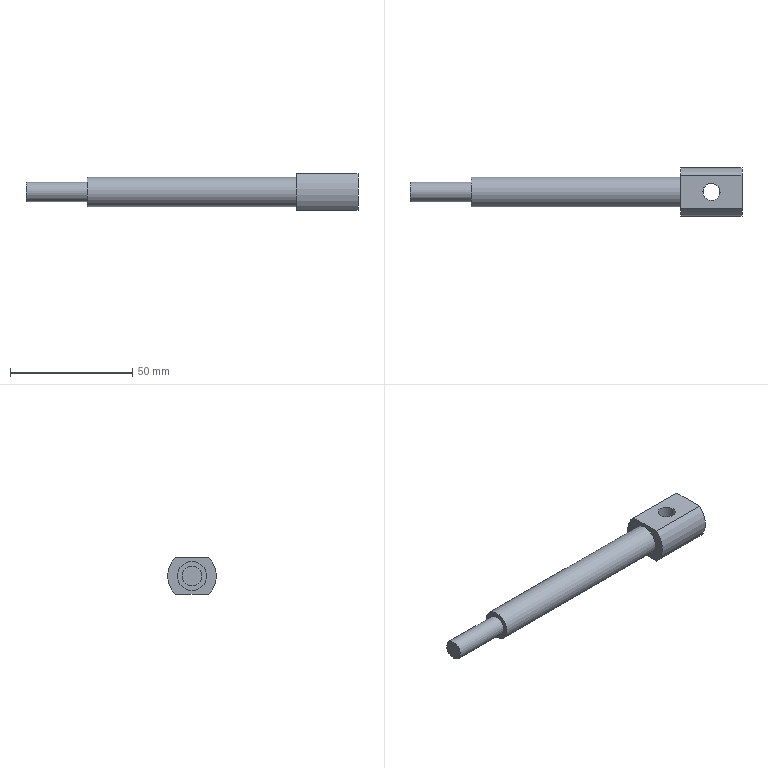Component | NX | LOCKING_SHAFT_2 | 1 solid | 11 faces | box 136 x 20 x 15 mm | volume 17126 mm3 | plane 6 | cylinder 5 | commonest cylinder face diameters 20 x2 12 x1 8 x1 7 x1
STEP:
#1=CARTESIAN_POINT('',(0.,0.,0.));
#2=DIRECTION('',(0.,0.,1.));
#3=DIRECTION('',(1.,0.,0.));
#4=AXIS2_PLACEMENT_3D('',#1,#2,#3);
#5=CARTESIAN_POINT('',(13.092,273.621,195.845));
#6=VERTEX_POINT('',#5);
#7=CARTESIAN_POINT('',(13.092,273.621,201.845));
#8=DIRECTION('',(-1.,0.,0.));
#9=DIRECTION('',(0.,0.,-1.));
#10=AXIS2_PLACEMENT_3D('',#7,#8,#9);
#11=CIRCLE('',#10,6.);
#12=CARTESIAN_POINT('',(13.092,273.621,201.845));
#13=DIRECTION('',(-1.,0.,0.));
#14=DIRECTION('',(0.,0.,-1.));
#15=AXIS2_PLACEMENT_3D('',#12,#13,#14);
#16=PLANE('',#15);
#17=CARTESIAN_POINT('',(0.,0.));
#18=DIRECTION('',(1.,0.));
#19=AXIS2_PLACEMENT_2D('',#17,#18);
#20=CIRCLE('',#19,6.);
#21=(GEOMETRIC_REPRESENTATION_CONTEXT(2)PARAMETRIC_REPRESENTATION_CONTEXT()REPRESENTATION_CONTEXT('',''));
#22=DEFINITIONAL_REPRESENTATION('',(#20),#21);
#23=PCURVE('',#16,#22);
#24=CARTESIAN_POINT('',(13.092,273.621,201.845));
#25=DIRECTION('',(-1.,0.,0.));
#26=DIRECTION('',(0.,0.,-1.));
#27=AXIS2_PLACEMENT_3D('',#24,#25,#26);
#28=CYLINDRICAL_SURFACE('',#27,6.);
#29=CARTESIAN_POINT('',(0.,0.));
#30=DIRECTION('',(1.,0.));
#31=VECTOR('',#30,1.);
#32=LINE('',#29,#31);
#33=(GEOMETRIC_REPRESENTATION_CONTEXT(2)PARAMETRIC_REPRESENTATION_CONTEXT()REPRESENTATION_CONTEXT('',''));
#34=DEFINITIONAL_REPRESENTATION('',(#32),#33);
#35=PCURVE('',#28,#34);
#36=SURFACE_CURVE('',#11,(#23,#35),.PCURVE_S1.);
#37=EDGE_CURVE('',#6,#6,#36,.T.);
#38=ORIENTED_EDGE('',*,*,#37,.F.);
#39=EDGE_LOOP('',(#38));
#40=FACE_BOUND('',#39,.T.);
#41=CARTESIAN_POINT('',(13.092,267.006,209.345));
#42=VERTEX_POINT('',#41);
#43=CARTESIAN_POINT('',(13.092,267.006,194.345));
#44=VERTEX_POINT('',#43);
#45=CARTESIAN_POINT('',(13.092,273.621,201.845));
#46=DIRECTION('',(1.,0.,0.));
#47=DIRECTION('',(0.,0.,-1.));
#48=AXIS2_PLACEMENT_3D('',#45,#46,#47);
#49=CIRCLE('',#48,10.);
#50=CARTESIAN_POINT('',(10.,0.));
#51=CARTESIAN_POINT('',(10.,-17.321));
#52=CARTESIAN_POINT('',(-5.,-8.66));
#53=CARTESIAN_POINT('',(-20.,-0.));
#54=CARTESIAN_POINT('',(-5.,8.66));
#55=CARTESIAN_POINT('',(10.,17.321));
#56=CARTESIAN_POINT('',(10.,0.));
#57=(BOUNDED_CURVE()B_SPLINE_CURVE(2,(#50,#51,#52,#53,#54,#55,#56),.UNSPECIFIED.,.T.,.F.)B_SPLINE_CURVE_WITH_KNOTS((1,2,2,2,2,1),(-2.094,0.,2.094,4.189,6.283,8.378),.UNSPECIFIED.)CURVE()GEOMETRIC_REPRESENTATION_ITEM()RATIONAL_B_SPLINE_CURVE((1.,0.5,1.,0.5,1.,0.5,1.))REPRESENTATION_ITEM(''));
#58=(GEOMETRIC_REPRESENTATION_CONTEXT(2)PARAMETRIC_REPRESENTATION_CONTEXT()REPRESENTATION_CONTEXT('',''));
#59=DEFINITIONAL_REPRESENTATION('',(#57),#58);
#60=PCURVE('',#16,#59);
#61=CARTESIAN_POINT('',(38.092,273.621,201.845));
#62=DIRECTION('',(-1.,0.,0.));
#63=DIRECTION('',(0.,0.,-1.));
#64=AXIS2_PLACEMENT_3D('',#61,#62,#63);
#65=CYLINDRICAL_SURFACE('',#64,10.);
#66=CARTESIAN_POINT('',(6.283,25.));
#67=DIRECTION('',(-1.,0.));
#68=VECTOR('',#67,1.);
#69=LINE('',#66,#68);
#70=(GEOMETRIC_REPRESENTATION_CONTEXT(2)PARAMETRIC_REPRESENTATION_CONTEXT()REPRESENTATION_CONTEXT('',''));
#71=DEFINITIONAL_REPRESENTATION('',(#69),#70);
#72=PCURVE('',#65,#71);
#73=SURFACE_CURVE('',#49,(#60,#72),.PCURVE_S1.);
#74=EDGE_CURVE('',#42,#44,#73,.T.);
#75=ORIENTED_EDGE('',*,*,#74,.F.);
#76=CARTESIAN_POINT('',(13.092,280.235,209.345));
#77=VERTEX_POINT('',#76);
#78=CARTESIAN_POINT('',(13.092,273.621,209.345));
#79=DIRECTION('',(0.,1.,0.));
#80=VECTOR('',#79,1.);
#81=LINE('',#78,#80);
#82=CARTESIAN_POINT('',(-7.5,0.));
#83=DIRECTION('',(0.,-1.));
#84=VECTOR('',#83,1.);
#85=LINE('',#82,#84);
#86=(GEOMETRIC_REPRESENTATION_CONTEXT(2)PARAMETRIC_REPRESENTATION_CONTEXT()REPRESENTATION_CONTEXT('',''));
#87=DEFINITIONAL_REPRESENTATION('',(#85),#86);
#88=PCURVE('',#16,#87);
#89=CARTESIAN_POINT('',(38.092,273.621,209.345));
#90=DIRECTION('',(0.,0.,1.));
#91=DIRECTION('',(-1.,0.,0.));
#92=AXIS2_PLACEMENT_3D('',#89,#90,#91);
#93=PLANE('',#92);
#94=CARTESIAN_POINT('',(25.,0.));
#95=DIRECTION('',(0.,-1.));
#96=VECTOR('',#95,1.);
#97=LINE('',#94,#96);
#98=(GEOMETRIC_REPRESENTATION_CONTEXT(2)PARAMETRIC_REPRESENTATION_CONTEXT()REPRESENTATION_CONTEXT('',''));
#99=DEFINITIONAL_REPRESENTATION('',(#97),#98);
#100=PCURVE('',#93,#99);
#101=SURFACE_CURVE('',#81,(#88,#100),.PCURVE_S1.);
#102=EDGE_CURVE('',#42,#77,#101,.T.);
#103=ORIENTED_EDGE('',*,*,#102,.T.);
#104=CARTESIAN_POINT('',(13.092,280.235,194.345));
#105=VERTEX_POINT('',#104);
#106=CARTESIAN_POINT('',(13.092,273.621,201.845));
#107=DIRECTION('',(1.,0.,0.));
#108=DIRECTION('',(0.,0.,-1.));
#109=AXIS2_PLACEMENT_3D('',#106,#107,#108);
#110=CIRCLE('',#109,10.);
#111=CARTESIAN_POINT('',(10.,0.));
#112=CARTESIAN_POINT('',(10.,-17.321));
#113=CARTESIAN_POINT('',(-5.,-8.66));
#114=CARTESIAN_POINT('',(-20.,-0.));
#115=CARTESIAN_POINT('',(-5.,8.66));
#116=CARTESIAN_POINT('',(10.,17.321));
#117=CARTESIAN_POINT('',(10.,0.));
#118=(BOUNDED_CURVE()B_SPLINE_CURVE(2,(#111,#112,#113,#114,#115,#116,#117),.UNSPECIFIED.,.T.,.F.)B_SPLINE_CURVE_WITH_KNOTS((1,2,2,2,2,1),(-2.094,0.,2.094,4.189,6.283,8.378),.UNSPECIFIED.)CURVE()GEOMETRIC_REPRESENTATION_ITEM()RATIONAL_B_SPLINE_CURVE((1.,0.5,1.,0.5,1.,0.5,1.))REPRESENTATION_ITEM(''));
#119=(GEOMETRIC_REPRESENTATION_CONTEXT(2)PARAMETRIC_REPRESENTATION_CONTEXT()REPRESENTATION_CONTEXT('',''));
#120=DEFINITIONAL_REPRESENTATION('',(#118),#119);
#121=PCURVE('',#16,#120);
#122=CARTESIAN_POINT('',(38.092,273.621,201.845));
#123=DIRECTION('',(-1.,0.,0.));
#124=DIRECTION('',(0.,0.,-1.));
#125=AXIS2_PLACEMENT_3D('',#122,#123,#124);
#126=CYLINDRICAL_SURFACE('',#125,10.);
#127=CARTESIAN_POINT('',(6.283,25.));
#128=DIRECTION('',(-1.,0.));
#129=VECTOR('',#128,1.);
#130=LINE('',#127,#129);
#131=(GEOMETRIC_REPRESENTATION_CONTEXT(2)PARAMETRIC_REPRESENTATION_CONTEXT()REPRESENTATION_CONTEXT('',''));
#132=DEFINITIONAL_REPRESENTATION('',(#130),#131);
#133=PCURVE('',#126,#132);
#134=SURFACE_CURVE('',#110,(#121,#133),.PCURVE_S1.);
#135=EDGE_CURVE('',#105,#77,#134,.T.);
#136=ORIENTED_EDGE('',*,*,#135,.F.);
#137=CARTESIAN_POINT('',(13.092,273.621,194.345));
#138=DIRECTION('',(0.,-1.,0.));
#139=VECTOR('',#138,1.);
#140=LINE('',#137,#139);
#141=CARTESIAN_POINT('',(7.5,0.));
#142=DIRECTION('',(0.,1.));
#143=VECTOR('',#142,1.);
#144=LINE('',#141,#143);
#145=(GEOMETRIC_REPRESENTATION_CONTEXT(2)PARAMETRIC_REPRESENTATION_CONTEXT()REPRESENTATION_CONTEXT('',''));
#146=DEFINITIONAL_REPRESENTATION('',(#144),#145);
#147=PCURVE('',#16,#146);
#148=CARTESIAN_POINT('',(38.092,273.621,194.345));
#149=DIRECTION('',(0.,0.,-1.));
#150=DIRECTION('',(1.,0.,0.));
#151=AXIS2_PLACEMENT_3D('',#148,#149,#150);
#152=PLANE('',#151);
#153=CARTESIAN_POINT('',(-25.,0.));
#154=DIRECTION('',(0.,1.));
#155=VECTOR('',#154,1.);
#156=LINE('',#153,#155);
#157=(GEOMETRIC_REPRESENTATION_CONTEXT(2)PARAMETRIC_REPRESENTATION_CONTEXT()REPRESENTATION_CONTEXT('',''));
#158=DEFINITIONAL_REPRESENTATION('',(#156),#157);
#159=PCURVE('',#152,#158);
#160=SURFACE_CURVE('',#140,(#147,#159),.PCURVE_S1.);
#161=EDGE_CURVE('',#105,#44,#160,.T.);
#162=ORIENTED_EDGE('',*,*,#161,.T.);
#163=EDGE_LOOP('',(#75,#103,#136,#162));
#164=FACE_BOUND('',#163,.T.);
#165=ADVANCED_FACE('',(#40,#164),#16,.T.);
#166=CARTESIAN_POINT('',(38.092,280.235,209.345));
#167=VERTEX_POINT('',#166);
#168=CARTESIAN_POINT('',(38.092,280.235,194.345));
#169=VERTEX_POINT('',#168);
#170=CARTESIAN_POINT('',(38.092,273.621,201.845));
#171=DIRECTION('',(-1.,0.,0.));
#172=DIRECTION('',(0.,0.,-1.));
#173=AXIS2_PLACEMENT_3D('',#170,#171,#172);
#174=CIRCLE('',#173,10.);
#175=CARTESIAN_POINT('',(38.092,273.621,201.845));
#176=DIRECTION('',(1.,0.,0.));
#177=DIRECTION('',(0.,0.,1.));
#178=AXIS2_PLACEMENT_3D('',#175,#176,#177);
#179=PLANE('',#178);
#180=CARTESIAN_POINT('',(-10.,0.));
#181=CARTESIAN_POINT('',(-10.,17.321));
#182=CARTESIAN_POINT('',(5.,8.66));
#183=CARTESIAN_POINT('',(20.,0.));
#184=CARTESIAN_POINT('',(5.,-8.66));
#185=CARTESIAN_POINT('',(-10.,-17.321));
#186=CARTESIAN_POINT('',(-10.,0.));
#187=(BOUNDED_CURVE()B_SPLINE_CURVE(2,(#180,#181,#182,#183,#184,#185,#186),.UNSPECIFIED.,.T.,.F.)B_SPLINE_CURVE_WITH_KNOTS((1,2,2,2,2,1),(-2.094,0.,2.094,4.189,6.283,8.378),.UNSPECIFIED.)CURVE()GEOMETRIC_REPRESENTATION_ITEM()RATIONAL_B_SPLINE_CURVE((1.,0.5,1.,0.5,1.,0.5,1.))REPRESENTATION_ITEM(''));
#188=(GEOMETRIC_REPRESENTATION_CONTEXT(2)PARAMETRIC_REPRESENTATION_CONTEXT()REPRESENTATION_CONTEXT('',''));
#189=DEFINITIONAL_REPRESENTATION('',(#187),#188);
#190=PCURVE('',#179,#189);
#191=CARTESIAN_POINT('',(-0.,0.));
#192=DIRECTION('',(1.,0.));
#193=VECTOR('',#192,1.);
#194=LINE('',#191,#193);
#195=(GEOMETRIC_REPRESENTATION_CONTEXT(2)PARAMETRIC_REPRESENTATION_CONTEXT()REPRESENTATION_CONTEXT('',''));
#196=DEFINITIONAL_REPRESENTATION('',(#194),#195);
#197=PCURVE('',#126,#196);
#198=SURFACE_CURVE('',#174,(#190,#197),.PCURVE_S1.);
#199=EDGE_CURVE('',#167,#169,#198,.T.);
#200=ORIENTED_EDGE('',*,*,#199,.F.);
#201=CARTESIAN_POINT('',(38.092,267.006,209.345));
#202=VERTEX_POINT('',#201);
#203=CARTESIAN_POINT('',(38.092,273.621,209.345));
#204=DIRECTION('',(0.,-1.,0.));
#205=VECTOR('',#204,1.);
#206=LINE('',#203,#205);
#207=CARTESIAN_POINT('',(7.5,0.));
#208=DIRECTION('',(0.,1.));
#209=VECTOR('',#208,1.);
#210=LINE('',#207,#209);
#211=(GEOMETRIC_REPRESENTATION_CONTEXT(2)PARAMETRIC_REPRESENTATION_CONTEXT()REPRESENTATION_CONTEXT('',''));
#212=DEFINITIONAL_REPRESENTATION('',(#210),#211);
#213=PCURVE('',#179,#212);
#214=CARTESIAN_POINT('',(0.,0.));
#215=DIRECTION('',(0.,1.));
#216=VECTOR('',#215,1.);
#217=LINE('',#214,#216);
#218=(GEOMETRIC_REPRESENTATION_CONTEXT(2)PARAMETRIC_REPRESENTATION_CONTEXT()REPRESENTATION_CONTEXT('',''));
#219=DEFINITIONAL_REPRESENTATION('',(#217),#218);
#220=PCURVE('',#93,#219);
#221=SURFACE_CURVE('',#206,(#213,#220),.PCURVE_S1.);
#222=EDGE_CURVE('',#167,#202,#221,.T.);
#223=ORIENTED_EDGE('',*,*,#222,.T.);
#224=CARTESIAN_POINT('',(38.092,267.006,194.345));
#225=VERTEX_POINT('',#224);
#226=CARTESIAN_POINT('',(38.092,273.621,201.845));
#227=DIRECTION('',(-1.,0.,0.));
#228=DIRECTION('',(0.,0.,-1.));
#229=AXIS2_PLACEMENT_3D('',#226,#227,#228);
#230=CIRCLE('',#229,10.);
#231=CARTESIAN_POINT('',(-10.,0.));
#232=CARTESIAN_POINT('',(-10.,17.321));
#233=CARTESIAN_POINT('',(5.,8.66));
#234=CARTESIAN_POINT('',(20.,0.));
#235=CARTESIAN_POINT('',(5.,-8.66));
#236=CARTESIAN_POINT('',(-10.,-17.321));
#237=CARTESIAN_POINT('',(-10.,0.));
#238=(BOUNDED_CURVE()B_SPLINE_CURVE(2,(#231,#232,#233,#234,#235,#236,#237),.UNSPECIFIED.,.T.,.F.)B_SPLINE_CURVE_WITH_KNOTS((1,2,2,2,2,1),(-2.094,0.,2.094,4.189,6.283,8.378),.UNSPECIFIED.)CURVE()GEOMETRIC_REPRESENTATION_ITEM()RATIONAL_B_SPLINE_CURVE((1.,0.5,1.,0.5,1.,0.5,1.))REPRESENTATION_ITEM(''));
#239=(GEOMETRIC_REPRESENTATION_CONTEXT(2)PARAMETRIC_REPRESENTATION_CONTEXT()REPRESENTATION_CONTEXT('',''));
#240=DEFINITIONAL_REPRESENTATION('',(#238),#239);
#241=PCURVE('',#179,#240);
#242=CARTESIAN_POINT('',(0.,0.));
#243=DIRECTION('',(1.,0.));
#244=VECTOR('',#243,1.);
#245=LINE('',#242,#244);
#246=(GEOMETRIC_REPRESENTATION_CONTEXT(2)PARAMETRIC_REPRESENTATION_CONTEXT()REPRESENTATION_CONTEXT('',''));
#247=DEFINITIONAL_REPRESENTATION('',(#245),#246);
#248=PCURVE('',#65,#247);
#249=SURFACE_CURVE('',#230,(#241,#248),.PCURVE_S1.);
#250=EDGE_CURVE('',#225,#202,#249,.T.);
#251=ORIENTED_EDGE('',*,*,#250,.F.);
#252=CARTESIAN_POINT('',(38.092,273.621,194.345));
#253=DIRECTION('',(0.,1.,0.));
#254=VECTOR('',#253,1.);
#255=LINE('',#252,#254);
#256=CARTESIAN_POINT('',(-7.5,0.));
#257=DIRECTION('',(0.,-1.));
#258=VECTOR('',#257,1.);
#259=LINE('',#256,#258);
#260=(GEOMETRIC_REPRESENTATION_CONTEXT(2)PARAMETRIC_REPRESENTATION_CONTEXT()REPRESENTATION_CONTEXT('',''));
#261=DEFINITIONAL_REPRESENTATION('',(#259),#260);
#262=PCURVE('',#179,#261);
#263=CARTESIAN_POINT('',(0.,0.));
#264=DIRECTION('',(0.,-1.));
#265=VECTOR('',#264,1.);
#266=LINE('',#263,#265);
#267=(GEOMETRIC_REPRESENTATION_CONTEXT(2)PARAMETRIC_REPRESENTATION_CONTEXT()REPRESENTATION_CONTEXT('',''));
#268=DEFINITIONAL_REPRESENTATION('',(#266),#267);
#269=PCURVE('',#152,#268);
#270=SURFACE_CURVE('',#255,(#262,#269),.PCURVE_S1.);
#271=EDGE_CURVE('',#225,#169,#270,.T.);
#272=ORIENTED_EDGE('',*,*,#271,.T.);
#273=EDGE_LOOP('',(#200,#223,#251,#272));
#274=FACE_BOUND('',#273,.T.);
#275=ADVANCED_FACE('',(#274),#179,.T.);
#276=ORIENTED_EDGE('',*,*,#135,.T.);
#277=CARTESIAN_POINT('',(38.092,280.235,209.345));
#278=DIRECTION('',(1.,0.,0.));
#279=VECTOR('',#278,1.);
#280=LINE('',#277,#279);
#281=CARTESIAN_POINT('',(3.864,0.));
#282=DIRECTION('',(0.,-1.));
#283=VECTOR('',#282,1.);
#284=LINE('',#281,#283);
#285=(GEOMETRIC_REPRESENTATION_CONTEXT(2)PARAMETRIC_REPRESENTATION_CONTEXT()REPRESENTATION_CONTEXT('',''));
#286=DEFINITIONAL_REPRESENTATION('',(#284),#285);
#287=PCURVE('',#126,#286);
#288=CARTESIAN_POINT('',(0.,-6.614));
#289=DIRECTION('',(-1.,0.));
#290=VECTOR('',#289,1.);
#291=LINE('',#288,#290);
#292=(GEOMETRIC_REPRESENTATION_CONTEXT(2)PARAMETRIC_REPRESENTATION_CONTEXT()REPRESENTATION_CONTEXT('',''));
#293=DEFINITIONAL_REPRESENTATION('',(#291),#292);
#294=PCURVE('',#93,#293);
#295=SURFACE_CURVE('',#280,(#287,#294),.PCURVE_S1.);
#296=EDGE_CURVE('',#77,#167,#295,.T.);
#297=ORIENTED_EDGE('',*,*,#296,.T.);
#298=ORIENTED_EDGE('',*,*,#199,.T.);
#299=CARTESIAN_POINT('',(38.092,280.235,194.345));
#300=DIRECTION('',(-1.,0.,0.));
#301=VECTOR('',#300,1.);
#302=LINE('',#299,#301);
#303=CARTESIAN_POINT('',(5.56,0.));
#304=DIRECTION('',(0.,1.));
#305=VECTOR('',#304,1.);
#306=LINE('',#303,#305);
#307=(GEOMETRIC_REPRESENTATION_CONTEXT(2)PARAMETRIC_REPRESENTATION_CONTEXT()REPRESENTATION_CONTEXT('',''));
#308=DEFINITIONAL_REPRESENTATION('',(#306),#307);
#309=PCURVE('',#126,#308);
#310=CARTESIAN_POINT('',(0.,-6.614));
#311=DIRECTION('',(-1.,0.));
#312=VECTOR('',#311,1.);
#313=LINE('',#310,#312);
#314=(GEOMETRIC_REPRESENTATION_CONTEXT(2)PARAMETRIC_REPRESENTATION_CONTEXT()REPRESENTATION_CONTEXT('',''));
#315=DEFINITIONAL_REPRESENTATION('',(#313),#314);
#316=PCURVE('',#152,#315);
#317=SURFACE_CURVE('',#302,(#309,#316),.PCURVE_S1.);
#318=EDGE_CURVE('',#169,#105,#317,.T.);
#319=ORIENTED_EDGE('',*,*,#318,.T.);
#320=EDGE_LOOP('',(#276,#297,#298,#319));
#321=FACE_BOUND('',#320,.T.);
#322=ADVANCED_FACE('',(#321),#126,.T.);
#323=ORIENTED_EDGE('',*,*,#250,.T.);
#324=CARTESIAN_POINT('',(38.092,267.006,209.345));
#325=DIRECTION('',(-1.,0.,0.));
#326=VECTOR('',#325,1.);
#327=LINE('',#324,#326);
#328=CARTESIAN_POINT('',(2.419,0.));
#329=DIRECTION('',(0.,1.));
#330=VECTOR('',#329,1.);
#331=LINE('',#328,#330);
#332=(GEOMETRIC_REPRESENTATION_CONTEXT(2)PARAMETRIC_REPRESENTATION_CONTEXT()REPRESENTATION_CONTEXT('',''));
#333=DEFINITIONAL_REPRESENTATION('',(#331),#332);
#334=PCURVE('',#65,#333);
#335=CARTESIAN_POINT('',(0.,6.614));
#336=DIRECTION('',(1.,0.));
#337=VECTOR('',#336,1.);
#338=LINE('',#335,#337);
#339=(GEOMETRIC_REPRESENTATION_CONTEXT(2)PARAMETRIC_REPRESENTATION_CONTEXT()REPRESENTATION_CONTEXT('',''));
#340=DEFINITIONAL_REPRESENTATION('',(#338),#339);
#341=PCURVE('',#93,#340);
#342=SURFACE_CURVE('',#327,(#334,#341),.PCURVE_S1.);
#343=EDGE_CURVE('',#202,#42,#342,.T.);
#344=ORIENTED_EDGE('',*,*,#343,.T.);
#345=ORIENTED_EDGE('',*,*,#74,.T.);
#346=CARTESIAN_POINT('',(38.092,267.006,194.345));
#347=DIRECTION('',(1.,0.,0.));
#348=VECTOR('',#347,1.);
#349=LINE('',#346,#348);
#350=CARTESIAN_POINT('',(0.7227,0.));
#351=DIRECTION('',(0.,-1.));
#352=VECTOR('',#351,1.);
#353=LINE('',#350,#352);
#354=(GEOMETRIC_REPRESENTATION_CONTEXT(2)PARAMETRIC_REPRESENTATION_CONTEXT()REPRESENTATION_CONTEXT('',''));
#355=DEFINITIONAL_REPRESENTATION('',(#353),#354);
#356=PCURVE('',#65,#355);
#357=CARTESIAN_POINT('',(0.,6.614));
#358=DIRECTION('',(1.,0.));
#359=VECTOR('',#358,1.);
#360=LINE('',#357,#359);
#361=(GEOMETRIC_REPRESENTATION_CONTEXT(2)PARAMETRIC_REPRESENTATION_CONTEXT()REPRESENTATION_CONTEXT('',''));
#362=DEFINITIONAL_REPRESENTATION('',(#360),#361);
#363=PCURVE('',#152,#362);
#364=SURFACE_CURVE('',#349,(#356,#363),.PCURVE_S1.);
#365=EDGE_CURVE('',#44,#225,#364,.T.);
#366=ORIENTED_EDGE('',*,*,#365,.T.);
#367=EDGE_LOOP('',(#323,#344,#345,#366));
#368=FACE_BOUND('',#367,.T.);
#369=ADVANCED_FACE('',(#368),#65,.T.);
#370=CARTESIAN_POINT('',(25.592,270.121,194.345));
#371=VERTEX_POINT('',#370);
#372=CARTESIAN_POINT('',(25.592,273.621,194.345));
#373=DIRECTION('',(0.,0.,-1.));
#374=DIRECTION('',(0.,-1.,0.));
#375=AXIS2_PLACEMENT_3D('',#372,#373,#374);
#376=CIRCLE('',#375,3.5);
#377=CARTESIAN_POINT('',(-12.5,0.));
#378=DIRECTION('',(0.,1.));
#379=AXIS2_PLACEMENT_2D('',#377,#378);
#380=CIRCLE('',#379,3.5);
#381=(GEOMETRIC_REPRESENTATION_CONTEXT(2)PARAMETRIC_REPRESENTATION_CONTEXT()REPRESENTATION_CONTEXT('',''));
#382=DEFINITIONAL_REPRESENTATION('',(#380),#381);
#383=PCURVE('',#152,#382);
#384=CARTESIAN_POINT('',(25.592,273.621,211.345));
#385=DIRECTION('',(0.,0.,-1.));
#386=DIRECTION('',(1.,0.,0.));
#387=AXIS2_PLACEMENT_3D('',#384,#385,#386);
#388=CYLINDRICAL_SURFACE('',#387,3.5);
#389=CARTESIAN_POINT('',(1.571,17.));
#390=DIRECTION('',(1.,0.));
#391=VECTOR('',#390,1.);
#392=LINE('',#389,#391);
#393=(GEOMETRIC_REPRESENTATION_CONTEXT(2)PARAMETRIC_REPRESENTATION_CONTEXT()REPRESENTATION_CONTEXT('',''));
#394=DEFINITIONAL_REPRESENTATION('',(#392),#393);
#395=PCURVE('',#388,#394);
#396=SURFACE_CURVE('',#376,(#383,#395),.PCURVE_S1.);
#397=EDGE_CURVE('',#371,#371,#396,.T.);
#398=ORIENTED_EDGE('',*,*,#397,.F.);
#399=EDGE_LOOP('',(#398));
#400=FACE_BOUND('',#399,.T.);
#401=ORIENTED_EDGE('',*,*,#365,.F.);
#402=ORIENTED_EDGE('',*,*,#161,.F.);
#403=ORIENTED_EDGE('',*,*,#318,.F.);
#404=ORIENTED_EDGE('',*,*,#271,.F.);
#405=EDGE_LOOP('',(#401,#402,#403,#404));
#406=FACE_BOUND('',#405,.T.);
#407=ADVANCED_FACE('',(#400,#406),#152,.T.);
#408=CARTESIAN_POINT('',(22.092,273.621,209.345));
#409=VERTEX_POINT('',#408);
#410=CARTESIAN_POINT('',(25.592,270.121,209.345));
#411=VERTEX_POINT('',#410);
#412=CARTESIAN_POINT('',(25.592,273.621,209.345));
#413=DIRECTION('',(0.,0.,1.));
#414=DIRECTION('',(-1.,0.,0.));
#415=AXIS2_PLACEMENT_3D('',#412,#413,#414);
#416=CIRCLE('',#415,3.5);
#417=CARTESIAN_POINT('',(12.5,0.));
#418=DIRECTION('',(1.,0.));
#419=AXIS2_PLACEMENT_2D('',#417,#418);
#420=CIRCLE('',#419,3.5);
#421=(GEOMETRIC_REPRESENTATION_CONTEXT(2)PARAMETRIC_REPRESENTATION_CONTEXT()REPRESENTATION_CONTEXT('',''));
#422=DEFINITIONAL_REPRESENTATION('',(#420),#421);
#423=PCURVE('',#93,#422);
#424=CARTESIAN_POINT('',(3.142,2.));
#425=DIRECTION('',(-1.,0.));
#426=VECTOR('',#425,1.);
#427=LINE('',#424,#426);
#428=(GEOMETRIC_REPRESENTATION_CONTEXT(2)PARAMETRIC_REPRESENTATION_CONTEXT()REPRESENTATION_CONTEXT('',''));
#429=DEFINITIONAL_REPRESENTATION('',(#427),#428);
#430=PCURVE('',#388,#429);
#431=SURFACE_CURVE('',#416,(#423,#430),.PCURVE_S1.);
#432=EDGE_CURVE('',#409,#411,#431,.T.);
#433=ORIENTED_EDGE('',*,*,#432,.F.);
#434=CARTESIAN_POINT('',(25.592,273.621,209.345));
#435=DIRECTION('',(0.,0.,1.));
#436=DIRECTION('',(-1.,0.,0.));
#437=AXIS2_PLACEMENT_3D('',#434,#435,#436);
#438=CIRCLE('',#437,3.5);
#439=CARTESIAN_POINT('',(12.5,0.));
#440=DIRECTION('',(1.,0.));
#441=AXIS2_PLACEMENT_2D('',#439,#440);
#442=CIRCLE('',#441,3.5);
#443=(GEOMETRIC_REPRESENTATION_CONTEXT(2)PARAMETRIC_REPRESENTATION_CONTEXT()REPRESENTATION_CONTEXT('',''));
#444=DEFINITIONAL_REPRESENTATION('',(#442),#443);
#445=PCURVE('',#93,#444);
#446=CARTESIAN_POINT('',(9.425,2.));
#447=DIRECTION('',(-1.,0.));
#448=VECTOR('',#447,1.);
#449=LINE('',#446,#448);
#450=(GEOMETRIC_REPRESENTATION_CONTEXT(2)PARAMETRIC_REPRESENTATION_CONTEXT()REPRESENTATION_CONTEXT('',''));
#451=DEFINITIONAL_REPRESENTATION('',(#449),#450);
#452=PCURVE('',#388,#451);
#453=SURFACE_CURVE('',#438,(#445,#452),.PCURVE_S1.);
#454=EDGE_CURVE('',#411,#409,#453,.T.);
#455=ORIENTED_EDGE('',*,*,#454,.F.);
#456=EDGE_LOOP('',(#433,#455));
#457=FACE_BOUND('',#456,.T.);
#458=ORIENTED_EDGE('',*,*,#296,.F.);
#459=ORIENTED_EDGE('',*,*,#102,.F.);
#460=ORIENTED_EDGE('',*,*,#343,.F.);
#461=ORIENTED_EDGE('',*,*,#222,.F.);
#462=EDGE_LOOP('',(#458,#459,#460,#461));
#463=FACE_BOUND('',#462,.T.);
#464=ADVANCED_FACE('',(#457,#463),#93,.T.);
#465=CARTESIAN_POINT('',(-72.908,273.621,197.845));
#466=VERTEX_POINT('',#465);
#467=CARTESIAN_POINT('',(-72.908,273.621,201.845));
#468=DIRECTION('',(-1.,0.,0.));
#469=DIRECTION('',(0.,0.,-1.));
#470=AXIS2_PLACEMENT_3D('',#467,#468,#469);
#471=CIRCLE('',#470,4.);
#472=CARTESIAN_POINT('',(-72.908,273.621,201.845));
#473=DIRECTION('',(-1.,0.,0.));
#474=DIRECTION('',(0.,0.,-1.));
#475=AXIS2_PLACEMENT_3D('',#472,#473,#474);
#476=PLANE('',#475);
#477=CARTESIAN_POINT('',(0.,0.));
#478=DIRECTION('',(1.,0.));
#479=AXIS2_PLACEMENT_2D('',#477,#478);
#480=CIRCLE('',#479,4.);
#481=(GEOMETRIC_REPRESENTATION_CONTEXT(2)PARAMETRIC_REPRESENTATION_CONTEXT()REPRESENTATION_CONTEXT('',''));
#482=DEFINITIONAL_REPRESENTATION('',(#480),#481);
#483=PCURVE('',#476,#482);
#484=CARTESIAN_POINT('',(-72.908,273.621,201.845));
#485=DIRECTION('',(-1.,0.,0.));
#486=DIRECTION('',(0.,0.,-1.));
#487=AXIS2_PLACEMENT_3D('',#484,#485,#486);
#488=CYLINDRICAL_SURFACE('',#487,4.);
#489=CARTESIAN_POINT('',(0.,0.));
#490=DIRECTION('',(1.,0.));
#491=VECTOR('',#490,1.);
#492=LINE('',#489,#491);
#493=(GEOMETRIC_REPRESENTATION_CONTEXT(2)PARAMETRIC_REPRESENTATION_CONTEXT()REPRESENTATION_CONTEXT('',''));
#494=DEFINITIONAL_REPRESENTATION('',(#492),#493);
#495=PCURVE('',#488,#494);
#496=SURFACE_CURVE('',#471,(#483,#495),.PCURVE_S1.);
#497=EDGE_CURVE('',#466,#466,#496,.T.);
#498=ORIENTED_EDGE('',*,*,#497,.F.);
#499=EDGE_LOOP('',(#498));
#500=FACE_BOUND('',#499,.T.);
#501=CARTESIAN_POINT('',(-72.908,273.621,195.845));
#502=VERTEX_POINT('',#501);
#503=CARTESIAN_POINT('',(-72.908,273.621,201.845));
#504=DIRECTION('',(1.,0.,0.));
#505=DIRECTION('',(0.,0.,-1.));
#506=AXIS2_PLACEMENT_3D('',#503,#504,#505);
#507=CIRCLE('',#506,6.);
#508=CARTESIAN_POINT('',(6.,0.));
#509=CARTESIAN_POINT('',(6.,-10.392));
#510=CARTESIAN_POINT('',(-3.,-5.196));
#511=CARTESIAN_POINT('',(-12.,-0.));
#512=CARTESIAN_POINT('',(-3.,5.196));
#513=CARTESIAN_POINT('',(6.,10.392));
#514=CARTESIAN_POINT('',(6.,0.));
#515=(BOUNDED_CURVE()B_SPLINE_CURVE(2,(#508,#509,#510,#511,#512,#513,#514),.UNSPECIFIED.,.T.,.F.)B_SPLINE_CURVE_WITH_KNOTS((1,2,2,2,2,1),(-2.094,0.,2.094,4.189,6.283,8.378),.UNSPECIFIED.)CURVE()GEOMETRIC_REPRESENTATION_ITEM()RATIONAL_B_SPLINE_CURVE((1.,0.5,1.,0.5,1.,0.5,1.))REPRESENTATION_ITEM(''));
#516=(GEOMETRIC_REPRESENTATION_CONTEXT(2)PARAMETRIC_REPRESENTATION_CONTEXT()REPRESENTATION_CONTEXT('',''));
#517=DEFINITIONAL_REPRESENTATION('',(#515),#516);
#518=PCURVE('',#476,#517);
#519=CARTESIAN_POINT('',(6.283,86.));
#520=DIRECTION('',(-1.,0.));
#521=VECTOR('',#520,1.);
#522=LINE('',#519,#521);
#523=(GEOMETRIC_REPRESENTATION_CONTEXT(2)PARAMETRIC_REPRESENTATION_CONTEXT()REPRESENTATION_CONTEXT('',''));
#524=DEFINITIONAL_REPRESENTATION('',(#522),#523);
#525=PCURVE('',#28,#524);
#526=SURFACE_CURVE('',#507,(#518,#525),.PCURVE_S1.);
#527=EDGE_CURVE('',#502,#502,#526,.T.);
#528=ORIENTED_EDGE('',*,*,#527,.F.);
#529=EDGE_LOOP('',(#528));
#530=FACE_BOUND('',#529,.T.);
#531=ADVANCED_FACE('',(#500,#530),#476,.T.);
#532=ORIENTED_EDGE('',*,*,#527,.T.);
#533=CARTESIAN_POINT('',(13.092,273.621,195.845));
#534=CARTESIAN_POINT('',(-72.908,273.621,195.845));
#535=B_SPLINE_CURVE_WITH_KNOTS('',1,(#533,#534),.UNSPECIFIED.,.F.,.F.,(2,2),(0.,86.),.PIECEWISE_BEZIER_KNOTS.);
#536=CARTESIAN_POINT('',(0.,0.));
#537=DIRECTION('',(0.,1.));
#538=VECTOR('',#537,1.);
#539=LINE('',#536,#538);
#540=(GEOMETRIC_REPRESENTATION_CONTEXT(2)PARAMETRIC_REPRESENTATION_CONTEXT()REPRESENTATION_CONTEXT('',''));
#541=DEFINITIONAL_REPRESENTATION('',(#539),#540);
#542=PCURVE('',#28,#541);
#543=CARTESIAN_POINT('',(6.283,0.));
#544=DIRECTION('',(0.,1.));
#545=VECTOR('',#544,1.);
#546=LINE('',#543,#545);
#547=(GEOMETRIC_REPRESENTATION_CONTEXT(2)PARAMETRIC_REPRESENTATION_CONTEXT()REPRESENTATION_CONTEXT('',''));
#548=DEFINITIONAL_REPRESENTATION('',(#546),#547);
#549=PCURVE('',#28,#548);
#550=SEAM_CURVE('',#535,(#542,#549),.PCURVE_S1.);
#551=EDGE_CURVE('',#6,#502,#550,.T.);
#552=ORIENTED_EDGE('',*,*,#551,.F.);
#553=ORIENTED_EDGE('',*,*,#37,.T.);
#554=ORIENTED_EDGE('',*,*,#551,.T.);
#555=EDGE_LOOP('',(#532,#552,#553,#554));
#556=FACE_BOUND('',#555,.T.);
#557=ADVANCED_FACE('',(#556),#28,.T.);
#558=CARTESIAN_POINT('',(-97.908,273.621,197.845));
#559=VERTEX_POINT('',#558);
#560=CARTESIAN_POINT('',(-97.908,273.621,201.845));
#561=DIRECTION('',(1.,0.,0.));
#562=DIRECTION('',(0.,0.,-1.));
#563=AXIS2_PLACEMENT_3D('',#560,#561,#562);
#564=CIRCLE('',#563,4.);
#565=CARTESIAN_POINT('',(-97.908,273.621,201.845));
#566=DIRECTION('',(-1.,0.,0.));
#567=DIRECTION('',(0.,0.,-1.));
#568=AXIS2_PLACEMENT_3D('',#565,#566,#567);
#569=PLANE('',#568);
#570=CARTESIAN_POINT('',(4.,0.));
#571=CARTESIAN_POINT('',(4.,-6.928));
#572=CARTESIAN_POINT('',(-2.,-3.464));
#573=CARTESIAN_POINT('',(-8.,-0.));
#574=CARTESIAN_POINT('',(-2.,3.464));
#575=CARTESIAN_POINT('',(4.,6.928));
#576=CARTESIAN_POINT('',(4.,0.));
#577=(BOUNDED_CURVE()B_SPLINE_CURVE(2,(#570,#571,#572,#573,#574,#575,#576),.UNSPECIFIED.,.T.,.F.)B_SPLINE_CURVE_WITH_KNOTS((1,2,2,2,2,1),(-2.094,0.,2.094,4.189,6.283,8.378),.UNSPECIFIED.)CURVE()GEOMETRIC_REPRESENTATION_ITEM()RATIONAL_B_SPLINE_CURVE((1.,0.5,1.,0.5,1.,0.5,1.))REPRESENTATION_ITEM(''));
#578=(GEOMETRIC_REPRESENTATION_CONTEXT(2)PARAMETRIC_REPRESENTATION_CONTEXT()REPRESENTATION_CONTEXT('',''));
#579=DEFINITIONAL_REPRESENTATION('',(#577),#578);
#580=PCURVE('',#569,#579);
#581=CARTESIAN_POINT('',(6.283,25.));
#582=DIRECTION('',(-1.,0.));
#583=VECTOR('',#582,1.);
#584=LINE('',#581,#583);
#585=(GEOMETRIC_REPRESENTATION_CONTEXT(2)PARAMETRIC_REPRESENTATION_CONTEXT()REPRESENTATION_CONTEXT('',''));
#586=DEFINITIONAL_REPRESENTATION('',(#584),#585);
#587=PCURVE('',#488,#586);
#588=SURFACE_CURVE('',#564,(#580,#587),.PCURVE_S1.);
#589=EDGE_CURVE('',#559,#559,#588,.T.);
#590=ORIENTED_EDGE('',*,*,#589,.F.);
#591=EDGE_LOOP('',(#590));
#592=FACE_BOUND('',#591,.T.);
#593=ADVANCED_FACE('',(#592),#569,.T.);
#594=ORIENTED_EDGE('',*,*,#589,.T.);
#595=CARTESIAN_POINT('',(-72.908,273.621,197.845));
#596=CARTESIAN_POINT('',(-97.908,273.621,197.845));
#597=B_SPLINE_CURVE_WITH_KNOTS('',1,(#595,#596),.UNSPECIFIED.,.F.,.F.,(2,2),(0.,25.),.PIECEWISE_BEZIER_KNOTS.);
#598=CARTESIAN_POINT('',(0.,0.));
#599=DIRECTION('',(0.,1.));
#600=VECTOR('',#599,1.);
#601=LINE('',#598,#600);
#602=(GEOMETRIC_REPRESENTATION_CONTEXT(2)PARAMETRIC_REPRESENTATION_CONTEXT()REPRESENTATION_CONTEXT('',''));
#603=DEFINITIONAL_REPRESENTATION('',(#601),#602);
#604=PCURVE('',#488,#603);
#605=CARTESIAN_POINT('',(6.283,0.));
#606=DIRECTION('',(0.,1.));
#607=VECTOR('',#606,1.);
#608=LINE('',#605,#607);
#609=(GEOMETRIC_REPRESENTATION_CONTEXT(2)PARAMETRIC_REPRESENTATION_CONTEXT()REPRESENTATION_CONTEXT('',''));
#610=DEFINITIONAL_REPRESENTATION('',(#608),#609);
#611=PCURVE('',#488,#610);
#612=SEAM_CURVE('',#597,(#604,#611),.PCURVE_S1.);
#613=EDGE_CURVE('',#466,#559,#612,.T.);
#614=ORIENTED_EDGE('',*,*,#613,.F.);
#615=ORIENTED_EDGE('',*,*,#497,.T.);
#616=ORIENTED_EDGE('',*,*,#613,.T.);
#617=EDGE_LOOP('',(#594,#614,#615,#616));
#618=FACE_BOUND('',#617,.T.);
#619=ADVANCED_FACE('',(#618),#488,.T.);
#620=ORIENTED_EDGE('',*,*,#454,.F.);
#621=CARTESIAN_POINT('',(25.592,270.121,209.345));
#622=CARTESIAN_POINT('',(25.592,270.121,194.345));
#623=B_SPLINE_CURVE_WITH_KNOTS('',1,(#621,#622),.UNSPECIFIED.,.F.,.F.,(2,2),(2.,17.),.PIECEWISE_BEZIER_KNOTS.);
#624=CARTESIAN_POINT('',(7.854,0.));
#625=DIRECTION('',(0.,1.));
#626=VECTOR('',#625,1.);
#627=LINE('',#624,#626);
#628=(GEOMETRIC_REPRESENTATION_CONTEXT(2)PARAMETRIC_REPRESENTATION_CONTEXT()REPRESENTATION_CONTEXT('',''));
#629=DEFINITIONAL_REPRESENTATION('',(#627),#628);
#630=PCURVE('',#388,#629);
#631=CARTESIAN_POINT('',(1.571,0.));
#632=DIRECTION('',(0.,1.));
#633=VECTOR('',#632,1.);
#634=LINE('',#631,#633);
#635=(GEOMETRIC_REPRESENTATION_CONTEXT(2)PARAMETRIC_REPRESENTATION_CONTEXT()REPRESENTATION_CONTEXT('',''));
#636=DEFINITIONAL_REPRESENTATION('',(#634),#635);
#637=PCURVE('',#388,#636);
#638=SEAM_CURVE('',#623,(#630,#637),.PCURVE_S1.);
#639=EDGE_CURVE('',#411,#371,#638,.T.);
#640=ORIENTED_EDGE('',*,*,#639,.T.);
#641=ORIENTED_EDGE('',*,*,#397,.F.);
#642=ORIENTED_EDGE('',*,*,#639,.F.);
#643=ORIENTED_EDGE('',*,*,#432,.F.);
#644=EDGE_LOOP('',(#620,#640,#641,#642,#643));
#645=FACE_BOUND('',#644,.F.);
#646=ADVANCED_FACE('',(#645),#388,.F.);
#647=CLOSED_SHELL('',(#165,#275,#322,#369,#407,#464,#531,#557,#593,#619,#646));
#648=MANIFOLD_SOLID_BREP('',#647);
#649=(LENGTH_UNIT()NAMED_UNIT(*)SI_UNIT(.MILLI.,.METRE.));
#650=UNCERTAINTY_MEASURE_WITH_UNIT(LENGTH_MEASURE(0.000002),#649,'','');
#651=(NAMED_UNIT(*)PLANE_ANGLE_UNIT()SI_UNIT($,.RADIAN.));
#652=(NAMED_UNIT(*)SI_UNIT($,.STERADIAN.)SOLID_ANGLE_UNIT());
#653=(GEOMETRIC_REPRESENTATION_CONTEXT(3)GLOBAL_UNCERTAINTY_ASSIGNED_CONTEXT((#650))GLOBAL_UNIT_ASSIGNED_CONTEXT((#649,#651,#652))REPRESENTATION_CONTEXT('',''));
#654=ADVANCED_BREP_SHAPE_REPRESENTATION('',(#4,#648),#653);